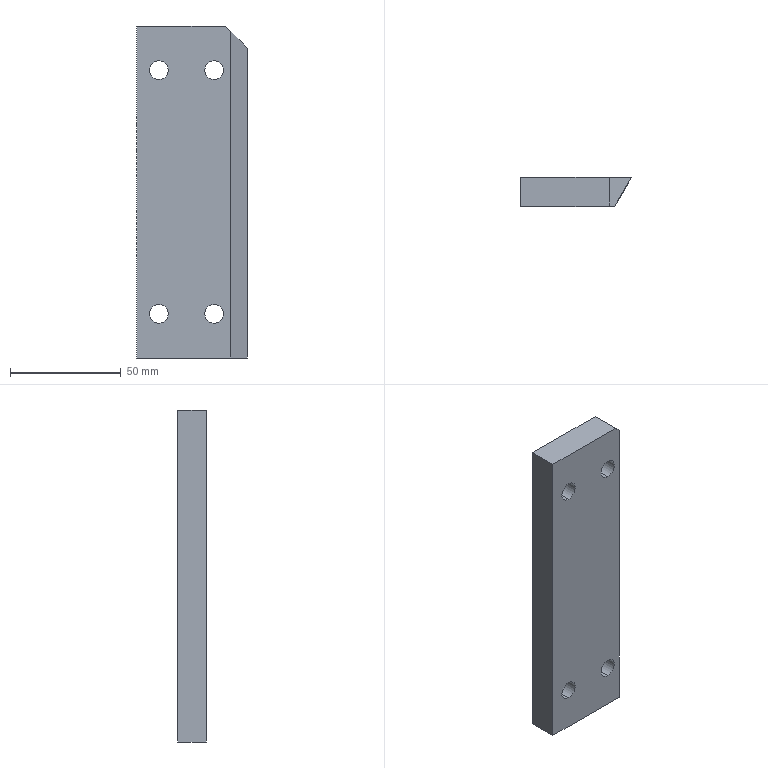CAM job | Mastercam | mm | 8 operations | part box 50 x 13 x 150
1. Facing | 20 - 63 平铣刀
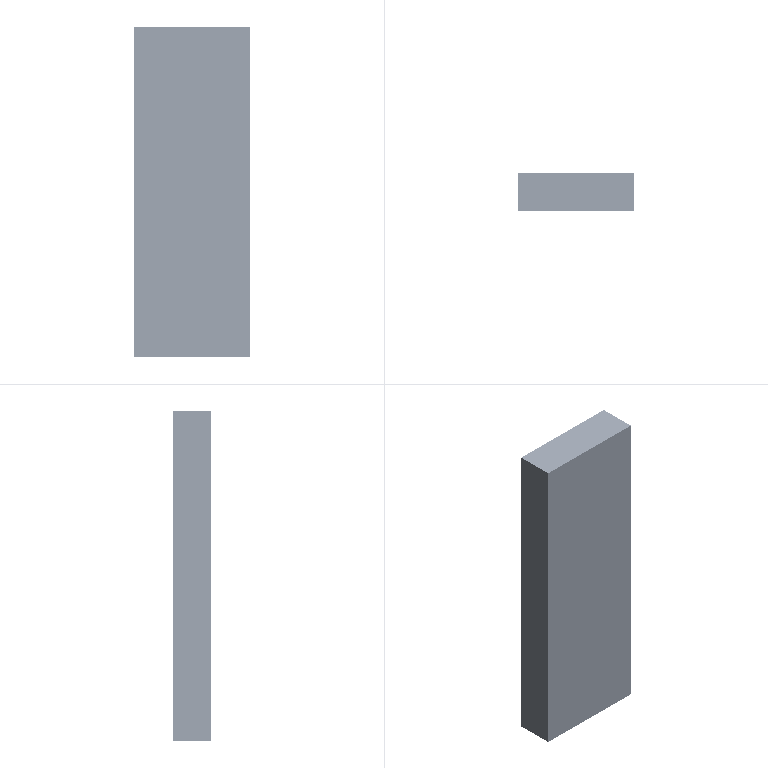2. 2D High Speed (2D Dynamic Mill) | 12 - 12 平铣刀
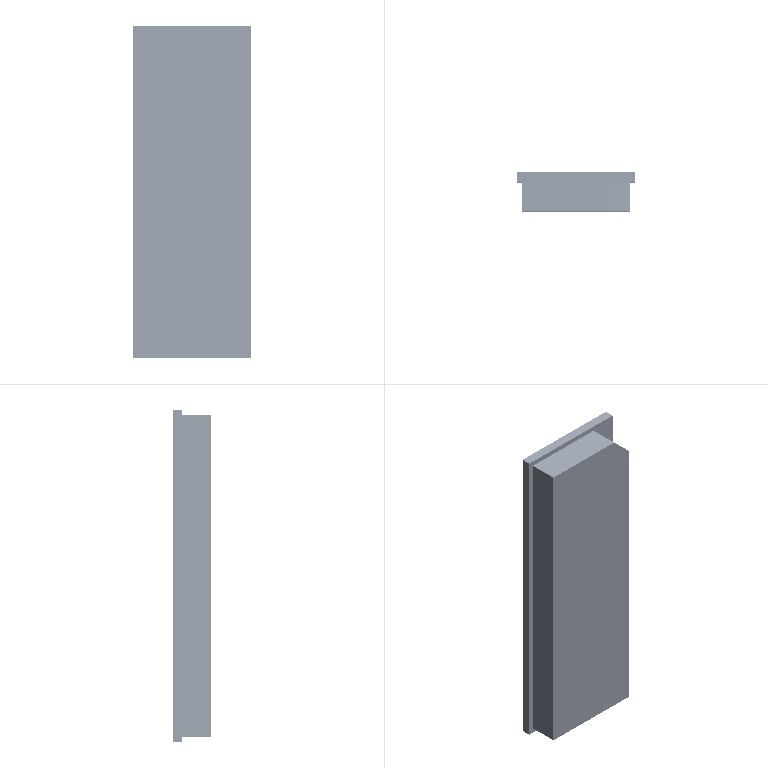3. Contour (2D) | 12 - 12 平铣刀
4. Drill/Counterbore | 7 - 4 倒角刀
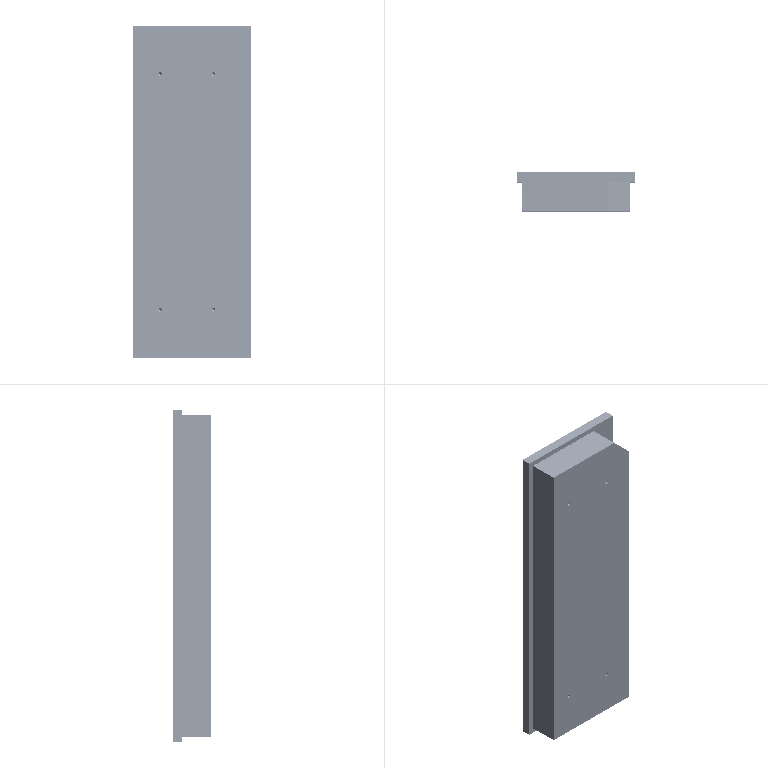5. Contour (2D chamfer) | 7 - 4 倒角刀
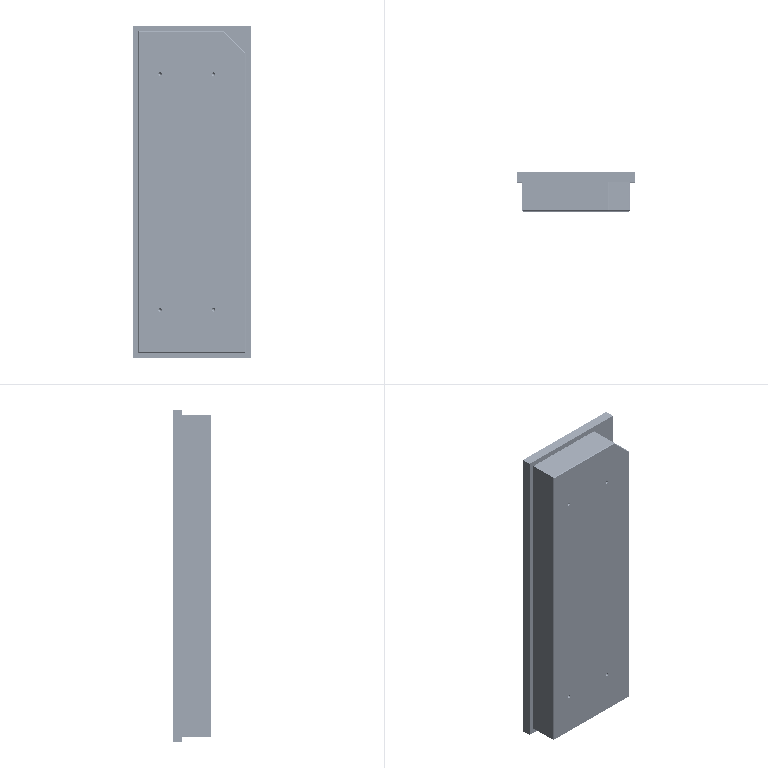6. Facing | 20 - 63 平铣刀
7. Contour (2D chamfer) | 7 - 4 倒角刀
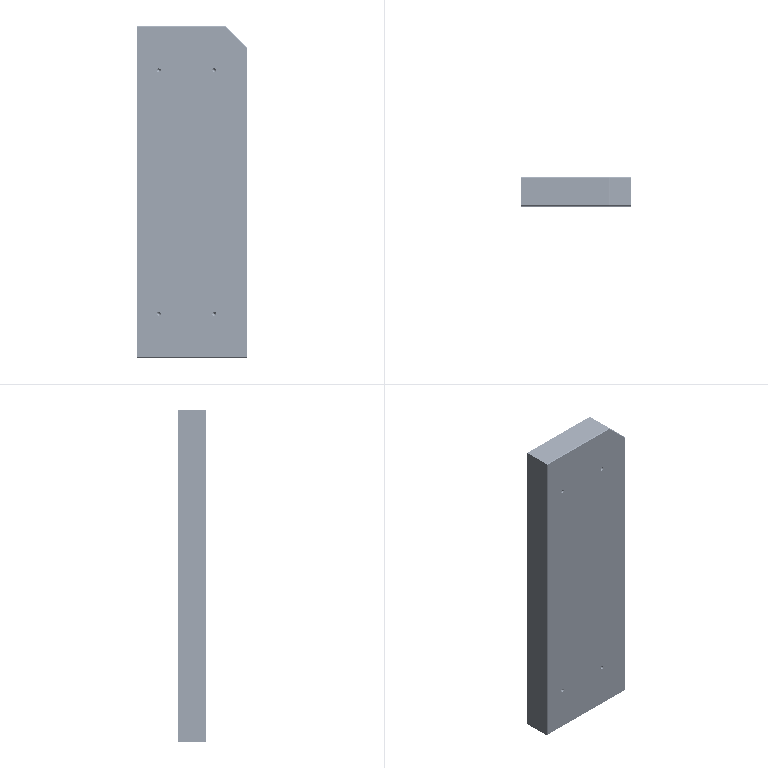8. Surface Finish Flowline | 9 - 8 圆鼻铣刀